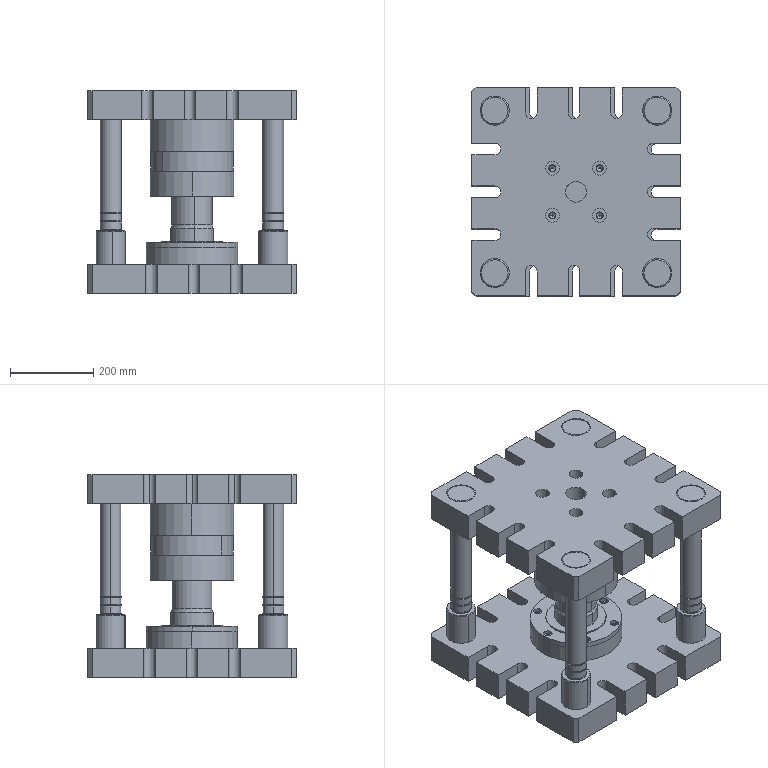Assembly | SolidWorks | mm | 38 component files | 39 solids | 1186 faces | box 500 x 500 x 486 mm | volume 41595547 mm3 | cylinder 539 | plane 439 | cone 134 | torus 74 | commonest cylinder face diameters 36 x64 50 x58 70 x32 48 x32 1.6 x32 3 x32 96 x31 28 x30
Bill of materials:
1 | 1 |  | Thick-walled plain cylindrical ring/spacer with a concentric through bore; height roughly half the outer diameter.
2 | 1 |  | Stepped cylindrical bushing with a through bore. It has a smaller upper body, a slightly larger lower body joined by a short tapered transition, a narrow relief groove or undercut just above the base, and a thin, wider flange at the bottom.
3 | 1 |  | Flat circular disc with a central internally toothed (spline- or gear-like) through opening and four small through holes equally spaced on a bolt circle near the rim.
5 | 1 |  | Thin-walled plain cylindrical ring or short tube with a large concentric through bore.
DieCore | 1 |  | Ring with a slightly tapered (conical) outer surface, wider at the top than at the bottom, and a concentric through bore.
DiePad | 1 |  | Thick cylindrical disc or hub with a central through bore and four small blind holes equally spaced on a bolt circle.
DieRetainingRing | 1 |  | Flat stepped annular washer/ring: a wider, thin base ring with a smaller-diameter raised ring on top, and a common through bore.
DieStressRing | 1 |  | Large cylindrical ring/collar with a big central bore and four small through holes equally spaced in the annular end face. A narrow internal step or ledge appears at the bore.
GuideBushing | 4 |  | Flanged cylindrical sleeve/bushing: a long tubular body with a through bore and a short, wider flange at one end, with small chamfers on the outer edges.
GuidePost | 4 |  | Solid headed pin: a long cylindrical shank with a short, wider, chamfered disc head at one end and several narrow circumferential grooves near the opposite end.
hexagon socket head cap screws gb | 16 |  | Socket-head screw-like part: a cylindrical head with a rounded top edge and a hexagonal socket recess, plus a plain cylindrical shank with a chamfered end. No thread is modeled.
LowerDiePlate | 1 |  | Square flat plate with small chamfered corners, four counterbored corner holes, twelve round-ended slots open to the edges (three per side), a central through hole, and four smaller through holes around it.
PunchMandrel | 1 |  | Stepped solid cylinder: a long, slender cylindrical shank with a short, larger-diameter coaxial collar at one end.
PunchPad | 1 |  | Plain solid circular disc: a short cylinder with flat parallel faces and no visible holes or features.
PunchRetainer | 1 |  | Thin flat annular ring (flange-like plate) with a large central bore and six small holes evenly spaced around a bolt circle.
UpperDieHolder | 1 |  | Thick annular ring with a large central bore and six small axial holes evenly spaced around the face.
UpperDiePlate | 1 |  | Square flat plate with chamfered corners, four large corner through holes, twelve U-shaped open slots around the edges, and a shallow central circular feature with eight small holes around it.
Mates:
1. coincident | DiePad-1 plane at (0, 0, 0) dir (0, 0, 1) | assembly plane at (0, 0, 0) dir (0, 0, 1)
2. coincident | DiePad-1 plane at (0, 0, 0) dir (0, 1, 0) | assembly plane at (0, 0, 0) dir (0, 1, 0)
3. coincident | DiePad-1 plane at (0, 0, 0) dir (1, 0, 0) | assembly plane at (0, 0, 0) dir (1, 0, 0)
4. concentric | DiePad-1 face at (0, 0, 80) dir (0, 0, -1) r 100 | LowerDiePlate-1 face at (0, 0, 145) dir (0, 0, -1) r 25
5. coincident | LowerDiePlate-1 plane at (0, 0, 75) dir (0, 1, 0) | assembly plane at (0, 0, 0) dir (0, 1, 0)
6. coincident | LowerDiePlate-1 face at (0, 0, 145) dir (0, 0, 1) | GuidePost-2 face at (-195, 195, 145) dir (0, 0, 1)
7. concentric | LowerDiePlate-1 face at (-195, 195, 125) dir (0, 0, 1) r 35 | GuidePost-2 face at (-195, 195, 125) dir (0, 0, -1) r 25
8. concentric | LowerDiePlate-1 face at (-195, -195, 125) dir (0, 0, 1) r 35 | GuidePost-1 face at (-195, -195, 125) dir (0, 0, -1) r 25
9. concentric | LowerDiePlate-1 face at (195, -195, 125) dir (0, 0, 1) r 35 | GuidePost-3 face at (195, -195, 125) dir (0, 0, -1) r 25
10. concentric | LowerDiePlate-1 face at (195, 195, 125) dir (0, 0, 1) r 35 | GuidePost-4 face at (195, 195, 125) dir (0, 0, -1) r 25
11. coincident | LowerDiePlate-1 face at (0, 0, 145) dir (0, 0, 1) | GuidePost-1 face at (-195, -195, 145) dir (0, 0, 1)
12. coincident | LowerDiePlate-1 face at (0, 0, 145) dir (0, 0, 1) | GuidePost-4 face at (195, 195, 145) dir (0, 0, 1)
13. coincident | LowerDiePlate-1 face at (0, 0, 145) dir (0, 0, 1) | GuidePost-3 face at (195, -195, 145) dir (0, 0, 1)
14. coincident | GuideBushing-3 face at (195, -195, -341) dir (0, 0, -1) | GuideBushing-4 face at (195, 195, -341) dir (0, 0, -1)
15. coincident | GuideBushing-2 face at (-195, 195, -341) dir (0, 0, -1) | GuideBushing-3 face at (195, -195, -341) dir (0, 0, -1)
16. coincident | GuideBushing-1 face at (-195, -195, -341) dir (0, 0, -1) | GuideBushing-2 face at (-195, 195, -341) dir (0, 0, -1)
17. concentric | GuideBushing-1 face at (-195, -195, -191) dir (0, 0, 1) r 35 | GuidePost-1 face at (-195, -195, 125) dir (0, 0, -1) r 25
18. concentric | GuidePost-2 face at (-195, 195, 125) dir (0, 0, -1) r 25 | GuideBushing-2 face at (-195, 195, -191) dir (0, 0, 1) r 35
19. concentric | GuidePost-3 face at (195, -195, 125) dir (0, 0, -1) r 25 | GuideBushing-3 face at (195, -195, -191) dir (0, 0, 1) r 35
20. concentric | GuidePost-4 face at (195, 195, 125) dir (0, 0, -1) r 25 | GuideBushing-4 face at (195, 195, -191) dir (0, 0, 1) r 35
21. coincident | DiePad-1 edge at (0, 0, 80) dir (0, 0, 1) r 100 | LowerDiePlate-1 face at (0, 0, 80) dir (0, 0, -1)
22. concentric | DieStressRing-1 face at (0, 0, -48) dir (0, 0, 1) r 100 | DieCore-1 edge at (0, 0, -108) dir (0, 0, -1) r 75.069
23. coincident | DieStressRing-1 face at (0, 0, -108) dir (0, 0, -1) | DieCore-1 face at (0, 55, -108) dir (0, 0, -1)
24. parallel | LowerDiePlate-1 face at (-250, -250, 145) dir (0, -1, 0) | DieCore-1 plane at (0, 0, -48) dir (0, 1, 0)
25. parallel | LowerDiePlate-1 face at (-250, -250, 145) dir (0, -1, 0) | DieStressRing-1 plane at (0, 0, -48) dir (0, 1, 0)
26. coincident | LowerDiePlate-1 face at (-250, 250, 145) dir (0, 1, 0) | UpperDiePlate-1 face at (250, 250, -341) dir (0, 1, 0)
27. coincident | LowerDiePlate-1 face at (-250, 250, 145) dir (-1, 0, 0) | UpperDiePlate-1 face at (-250, 250, -341) dir (-1, 0, 0)
28. coincident | GuideBushing-1 face at (-195, -195, -341) dir (0, 0, -1) | UpperDiePlate-1 face at (0, 0, -341) dir (0, 0, -1)
29. coincident | UpperDiePlate-1 face at (0, 0, -271) dir (0, 0, 1) | PunchPad-1 face at (0, 0, -271) dir (0, 0, -1)
30. concentric | DieCore-1 face at (0, 0, -109.661) dir (0, 0, -1) r 83.141 | PunchPad-1 face at (0, 0, -246) dir (0, 0, -1) r 82.5
31. distance | UpperDiePlate-1 face at (0, 0, -271) dir (0, 0, 1) | UpperDieHolder-1 face at (0, 0, -271) dir (0, 0, -1)
32. concentric | PunchPad-1 edge at (0, 0, -246) dir (0, 0, 1) r 82.5 | UpperDieHolder-1 face at (0, 0, -231) dir (0, 0, -1) r 110
33. parallel | UpperDiePlate-1 face at (250, 250, -341) dir (0, 1, 0) | UpperDieHolder-1 plane at (0, 0, -271) dir (0, 1, 0)
34. coincident | PunchPad-1 face at (0, 0, -246) dir (0, 0, 1) | DieRetainingRing-1 face at (0, 0, -246) dir (0, 0, -1)
35. concentric | UpperDieHolder-1 face at (0, 0, -231) dir (0, 0, -1) r 82.5 | DieRetainingRing-1 face at (0, 0, -216) dir (0, 0, 1) r 82.5
36. concentric | UpperDieHolder-1 face at (0, 0, -231) dir (0, 0, -1) r 110 | PunchRetainer-1 face at (0, 0, -219) dir (0, 0, -1) r 110
37. coincident | DieRetainingRing-1 face at (82.256, -6.346, -231) dir (0, 0, 1) | PunchRetainer-1 face at (0, 0, -231) dir (0, 0, -1)
38. concentric | PunchRetainer-1 face at (-95, 0, -219) dir (0, 0, -1) r 5.5 | hexagon socket head cap screws gb-11 face at (-95, 0, -232) dir (0, 0, 1) r 0.8
39. coincident | PunchRetainer-1 face at (-95, 0, -226) dir (0, 0, 1) | hexagon socket head cap screws gb-11 face at (-95, 0, -226) dir (0, 0, -1)
40. concentric | UpperDiePlate-1 face at (-95, 0, -316) dir (0, 0, -1) r 10 | hexagon socket head cap screws gb-12 face at (-95, 0, -310) dir (0, 0, -1) r 0.8
41. coincident | UpperDiePlate-1 face at (-95, 0, -316) dir (0, 0, -1) | hexagon socket head cap screws gb-12 face at (-95, 0, -316) dir (0, 0, 1)
42. concentric | DieStressRing-1 face at (0, 0, -48) dir (0, 0, 1) r 100 | 5-1 face at (0, 0, -48) dir (0, 0, -1) r 60
43. concentric | LowerDiePlate-1 face at (-56.569, 56.569, 145) dir (0, 0, -1) r 8.5 | hexagon socket head cap screws gb-1 face at (-56.569, 56.569, 109) dir (0, 0, 1) r 0.8
44. concentric | LowerDiePlate-1 face at (-56.569, -56.569, 145) dir (0, 0, -1) r 8.5 | hexagon socket head cap screws gb-4 face at (-56.569, -56.569, 109) dir (0, 0, 1) r 0.8
45. concentric | LowerDiePlate-1 face at (56.569, 56.569, 145) dir (0, 0, -1) r 8.5 | hexagon socket head cap screws gb-2 face at (56.569, 56.569, 109) dir (0, 0, 1) r 0.8
46. concentric | LowerDiePlate-1 face at (56.569, -56.569, 145) dir (0, 0, -1) r 8.5 | hexagon socket head cap screws gb-3 face at (56.569, -56.569, 109) dir (0, 0, 1) r 0.8
47. coincident | hexagon socket head cap screws gb-1 face at (-56.569, 56.569, 116.6) dir (0, 0, 1) | hexagon socket head cap screws gb-4 face at (-56.569, -56.569, 116.6) dir (0, 0, 1)
48. coincident | hexagon socket head cap screws gb-2 face at (56.569, 56.569, 116.6) dir (0, 0, 1) | hexagon socket head cap screws gb-3 face at (56.569, -56.569, 116.6) dir (0, 0, 1)
49. coincident | hexagon socket head cap screws gb-3 face at (56.569, -56.569, 116.6) dir (0, 0, 1) | hexagon socket head cap screws gb-4 face at (-56.569, -56.569, 116.6) dir (0, 0, 1)
50. coincident | LowerDiePlate-1 face at (-56.569, 56.569, 115) dir (0, 0, 1) | hexagon socket head cap screws gb-1 edge at (-56.569, 56.569, 115) dir (0, 0, -1) r 1.5
51. coincident | DiePad-1 face at (0, 0, 0) dir (0, 0, -1) | 3-1 face at (-45.962, 45.962, 0) dir (0, 0, 1)
52. coincident | DieCore-1 face at (0, 0, -48) dir (0, 0, 1) | 3-1 face at (-70.711, 70.711, -48) dir (0, 0, -1)
53. concentric | 1-1 face at (0, 0, -48) dir (0, 0, -1) r 48.03 | 5-1 face at (0, 0, -48) dir (0, 0, -1) r 48.03
54. coincident | 1-1 face at (0, 0, -48) dir (0, 0, 1) | 3-1 face at (0, 0, -48) dir (0, 0, -1)
55. concentric | PunchMandrel-1 face at (0, 0, -1) dir (0, 0, 1) r 26.825 | 2-1 face at (0, 0, -96) dir (0, 0, 1) r 48.025
56. coincident | DieRetainingRing-1 face at (54.837, -4.231, -231) dir (0, 0, -1) | 2-1 face at (-54.539, -7.105, -231) dir (0, 0, 1)
57. concentric | DieRetainingRing-1 face at (0, 0, -216) dir (0, 0, 1) r 55 | 2-1 face at (0, 0, -96) dir (0, 0, 1) r 51
58. coincident | PunchMandrel-1 face at (24.649, 17.535, -201) dir (0, 0, 1) | 2-1 face at (0, 0, -201) dir (0, 0, -1)
59. concentric | DieStressRing-1 face at (0, 0, -48) dir (0, 0, 1) r 100 | 3-1 face at (0, 0, -48) dir (0, 0, -1) r 100
60. concentric | DiePad-1 face at (0, 0, 80) dir (0, 0, -1) r 100 | 3-1 face at (0, 0, -48) dir (0, 0, -1) r 100
61. concentric | DieStressRing-1 face at (-87.5, 0, -78) dir (0, 0, -1) r 8.25 | 3-1 edge at (-87.5, 0, -48) dir (0, 0, 1) r 4.5